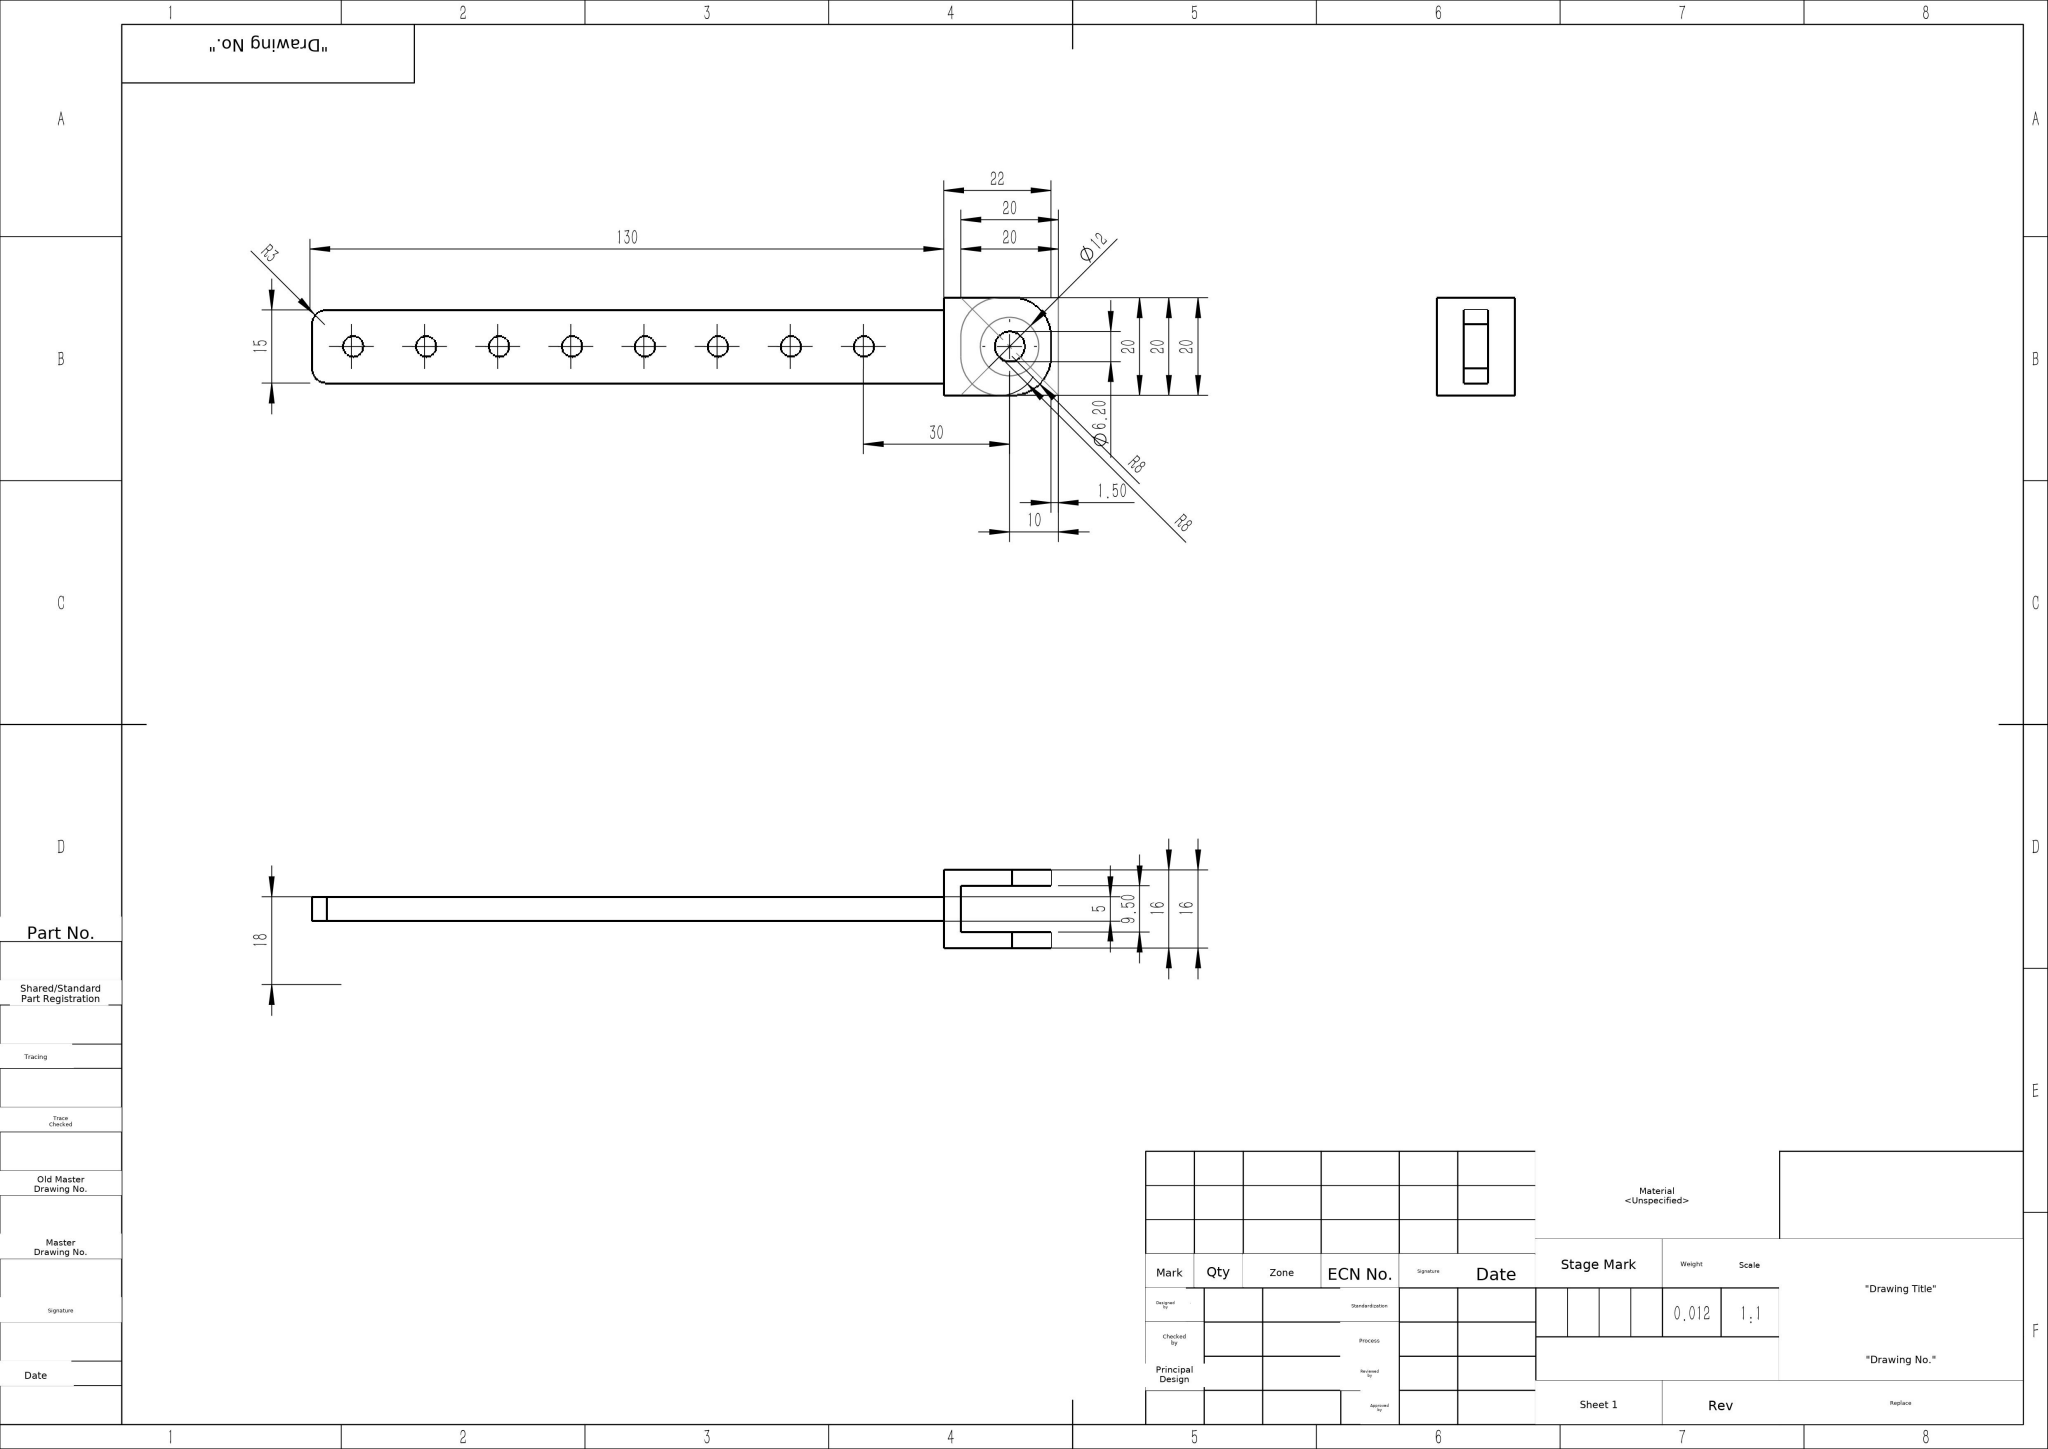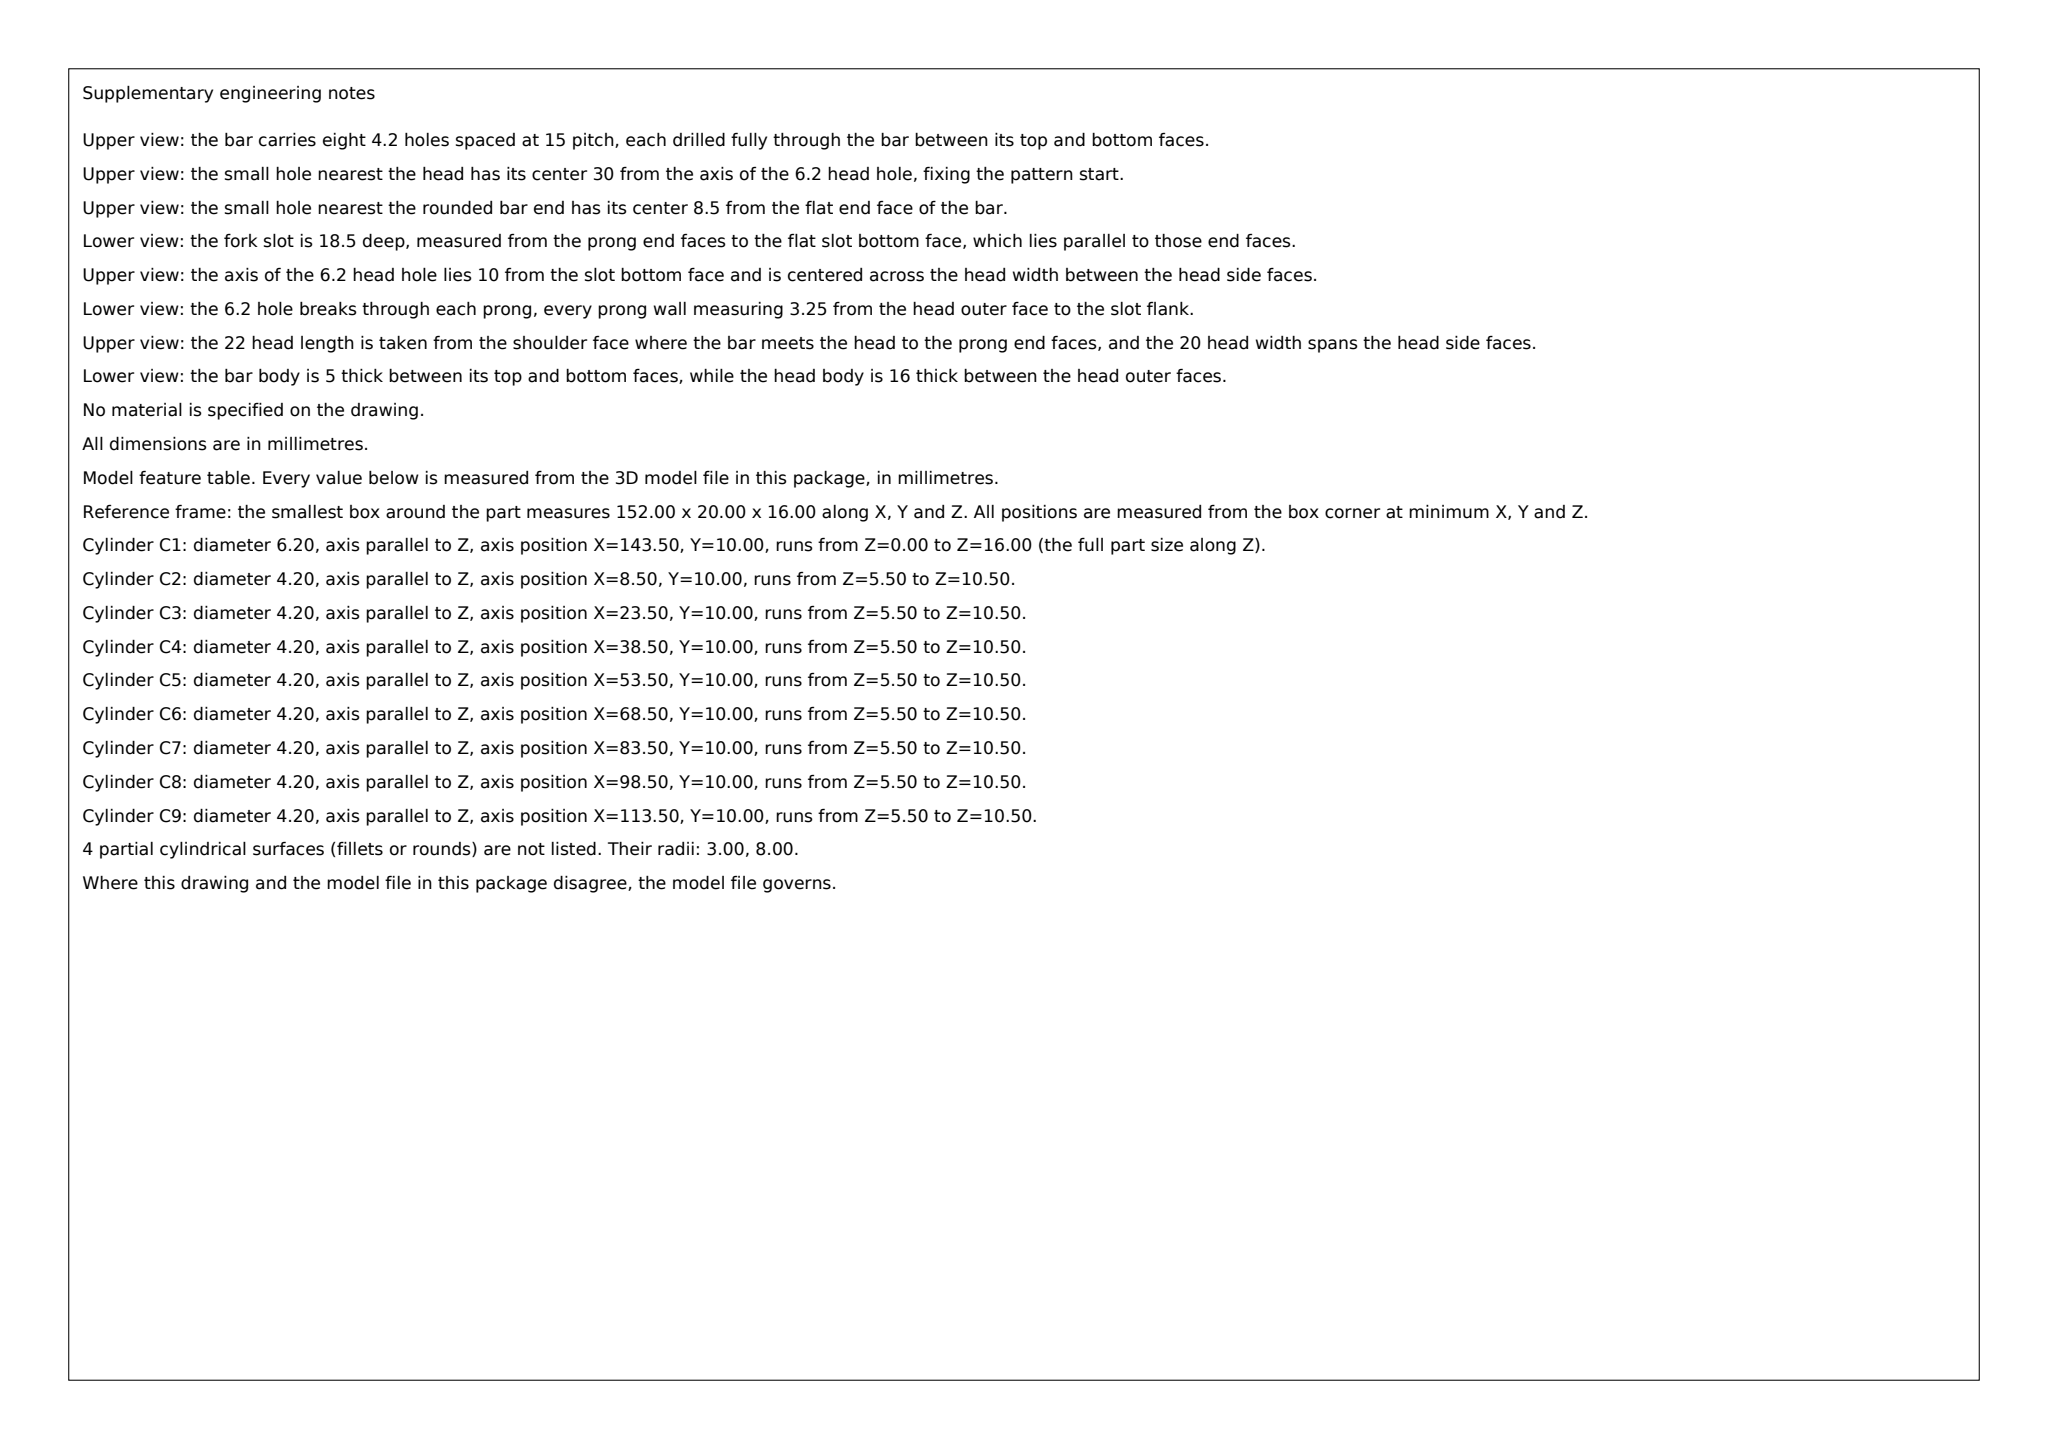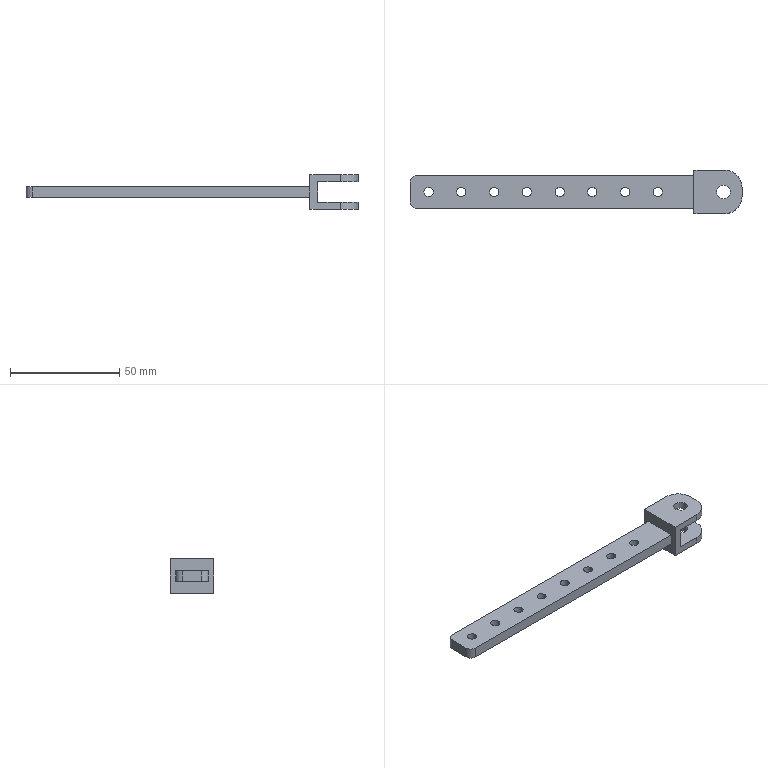Part | SolidWorks | mm | 1 solid | 41 faces | box 152 x 20 x 16 mm | volume 12327 mm3 | cylinder 26 | plane 15 | commonest cylinder face diameters 4.2 x16 6.2 x4 16 x4 6 x2
Drawing notes:
8X Ø4.20 PATTERN: 1ST HOLE CL 8.50 FROM LEFT END, 7X15 CHAIN | from the solid: 4.2 dia cyls at x=8.5,23.5,...,113.5; bar left face plane x=0.0
LAST Ø4.20 HOLE CL 16.50 FROM HEAD FACE (130 DIM FACE) | from the solid: last 4.2 hole x=113.5; plane x=130.0 -> 130-113.5=16.5
build123d program:
from build123d import *

# Parameters (mm, degrees)
SKETCH2_W           = 22
SKETCH2_H           = 20
BOSS_EXTRUDE2_DEPTH = 8
SKETCH3_W           = 20
SKETCH3_H           = 20
CUT_EXTRUDE1_DEPTH  = 4.75
SKETCH4_R           = 3.1
CUT_EXTRUDE3_DEPTH  = 16
SKETCH5_W           = 130
SKETCH5_H           = 15
BOSS_EXTRUDE3_DEPTH = 2.5
SKETCH6_R           = 2.1
CUT_EXTRUDE4_DEPTH  = 18
FILLET1_R           = 8
FILLET2_R           = 3


with BuildPart() as part:
    # Sketch2 → Boss-Extrude2 (new, symmetric)
    with BuildSketch(Plane.XY):
        with Locations((-2.5, 0)):
            Rectangle(SKETCH2_W, SKETCH2_H)
    extrude(amount=BOSS_EXTRUDE2_DEPTH, both=True)

    # Sketch3 → Cut-Extrude1 (cut, symmetric)
    with BuildSketch(Plane.XY):
        Rectangle(SKETCH3_W, SKETCH3_H)
    extrude(amount=CUT_EXTRUDE1_DEPTH, both=True, mode=Mode.SUBTRACT)

    # Sketch4 → Cut-Extrude3 (cut)
    with BuildSketch(Plane(origin=(0, 0, -8), x_dir=(-1, 0, 0), z_dir=(0, 0, -1))):
        Circle(SKETCH4_R)
    extrude(amount=-CUT_EXTRUDE3_DEPTH, mode=Mode.SUBTRACT)

    # Sketch5 → Boss-Extrude3 (add, symmetric)
    with BuildSketch(Plane.XY):
        with Locations((-78.5, 0)):
            Rectangle(SKETCH5_W, SKETCH5_H)
    extrude(amount=BOSS_EXTRUDE3_DEPTH, both=True)

    # Sketch6 → Cut-Extrude4 (cut)
    with BuildSketch(Plane(origin=(0, 0, -2.5), x_dir=(-1, 0, 0), z_dir=(0, 0, -1))):
        with Locations((30, 0)):
            Circle(SKETCH6_R)
        with Locations((45, 0)):
            Circle(SKETCH6_R)
        with Locations((60, 0)):
            Circle(SKETCH6_R)
        with Locations((75, 0)):
            Circle(SKETCH6_R)
        with Locations((90, 0)):
            Circle(SKETCH6_R)
        with Locations((105, 0)):
            Circle(SKETCH6_R)
        with Locations((120, 0)):
            Circle(SKETCH6_R)
        with Locations((135, 0)):
            Circle(SKETCH6_R)
    extrude(amount=-CUT_EXTRUDE4_DEPTH, mode=Mode.SUBTRACT)

    # Fillet1
    fillet1_edges = [part.edges().sort_by_distance(p)[0] for p in [
        (8.5, 10, -6.375),
        (8.5, -10, -6.375),
        (8.5, 10, 6.375),
        (8.5, -10, 6.375),
    ]]
    fillet(fillet1_edges, radius=FILLET1_R)

    # Fillet2
    fillet2_edges = [part.edges().sort_by_distance(p)[0] for p in [
        (-143.5, 7.5, 0),
        (-143.5, -7.5, 0),
    ]]
    fillet(fillet2_edges, radius=FILLET2_R)


solid = part.part